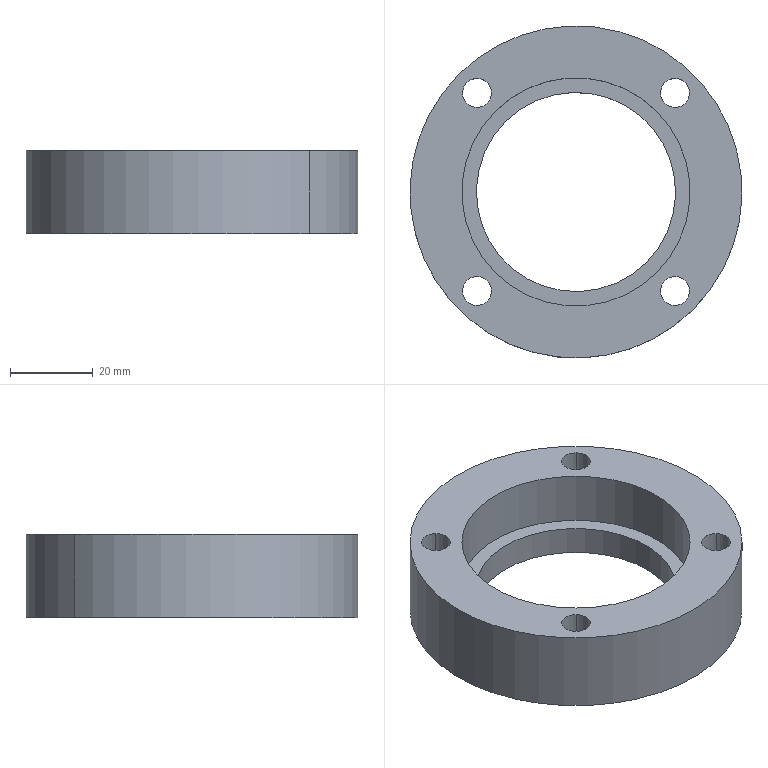Component | SolidWorks | 6006BearingHousing-3 | 1 solid | 29 faces | box 80 x 80 x 20 mm | volume 52542 mm3 | cylinder 22 | plane 7 | commonest cylinder face diameters 11 x8 7 x8 80 x2 55 x2 48 x2
STEP:
#1=COLOUR_RGB('',0.7922,0.8196,0.9333);
#2=FILL_AREA_STYLE_COLOUR('',#1);
#3=FILL_AREA_STYLE('',(#2));
#4=SURFACE_STYLE_FILL_AREA(#3);
#5=SURFACE_SIDE_STYLE('',(#4));
#6=SURFACE_STYLE_USAGE(.BOTH.,#5);
#7=PRESENTATION_STYLE_ASSIGNMENT((#6));
#8=CARTESIAN_POINT('',(7.284,48.013,-3.898));
#9=VERTEX_POINT('',#8);
#10=CARTESIAN_POINT('',(6.978,47.707,-3.898));
#11=VERTEX_POINT('',#10);
#12=CARTESIAN_POINT('',(7.131,47.86,-3.898));
#13=DIRECTION('',(0.,0.,-1.));
#14=DIRECTION('',(-0.7071,-0.7071,0.));
#15=AXIS2_PLACEMENT_3D('',#12,#13,#14);
#16=CIRCLE('',#15,0.2165);
#17=EDGE_CURVE('',#9,#11,#16,.T.);
#18=ORIENTED_EDGE('',*,*,#17,.F.);
#19=CARTESIAN_POINT('',(7.284,48.013,-4.134));
#20=VERTEX_POINT('',#19);
#21=CARTESIAN_POINT('',(7.284,48.013,-4.134));
#22=DIRECTION('',(0.,0.,-1.));
#23=VECTOR('',#22,39.37);
#24=LINE('',#21,#23);
#25=EDGE_CURVE('',#9,#20,#24,.T.);
#26=ORIENTED_EDGE('',*,*,#25,.T.);
#27=CARTESIAN_POINT('',(6.978,47.707,-4.134));
#28=VERTEX_POINT('',#27);
#29=CARTESIAN_POINT('',(7.131,47.86,-4.134));
#30=DIRECTION('',(0.,0.,-1.));
#31=DIRECTION('',(-0.7071,-0.7071,0.));
#32=AXIS2_PLACEMENT_3D('',#29,#30,#31);
#33=CIRCLE('',#32,0.2165);
#34=EDGE_CURVE('',#20,#28,#33,.T.);
#35=ORIENTED_EDGE('',*,*,#34,.T.);
#36=CARTESIAN_POINT('',(6.978,47.707,-4.134));
#37=DIRECTION('',(0.,0.,-1.));
#38=VECTOR('',#37,39.37);
#39=LINE('',#36,#38);
#40=EDGE_CURVE('',#11,#28,#39,.T.);
#41=ORIENTED_EDGE('',*,*,#40,.F.);
#42=EDGE_LOOP('',(#18,#26,#35,#41));
#43=FACE_OUTER_BOUND('',#42,.T.);
#44=CARTESIAN_POINT('',(7.131,47.86,-4.134));
#45=DIRECTION('',(0.,0.,-1.));
#46=DIRECTION('',(-0.7071,-0.7071,0.));
#47=AXIS2_PLACEMENT_3D('',#44,#45,#46);
#48=CYLINDRICAL_SURFACE('',#47,0.2165);
#49=ADVANCED_FACE('',(#43),#48,.F.);
#50=CARTESIAN_POINT('',(7.229,47.957,-3.346));
#51=VERTEX_POINT('',#50);
#52=CARTESIAN_POINT('',(7.034,47.762,-3.346));
#53=VERTEX_POINT('',#52);
#54=CARTESIAN_POINT('',(7.131,47.86,-3.346));
#55=DIRECTION('',(0.,0.,-1.));
#56=DIRECTION('',(-0.7071,-0.7071,0.));
#57=AXIS2_PLACEMENT_3D('',#54,#55,#56);
#58=CIRCLE('',#57,0.1378);
#59=EDGE_CURVE('',#51,#53,#58,.T.);
#60=ORIENTED_EDGE('',*,*,#59,.F.);
#61=CARTESIAN_POINT('',(7.229,47.957,-3.898));
#62=VERTEX_POINT('',#61);
#63=CARTESIAN_POINT('',(7.229,47.957,-4.134));
#64=DIRECTION('',(0.,0.,-1.));
#65=VECTOR('',#64,39.37);
#66=LINE('',#63,#65);
#67=EDGE_CURVE('',#51,#62,#66,.T.);
#68=ORIENTED_EDGE('',*,*,#67,.T.);
#69=CARTESIAN_POINT('',(7.034,47.762,-3.898));
#70=VERTEX_POINT('',#69);
#71=CARTESIAN_POINT('',(7.131,47.86,-3.898));
#72=DIRECTION('',(0.,0.,-1.));
#73=DIRECTION('',(-0.7071,-0.7071,0.));
#74=AXIS2_PLACEMENT_3D('',#71,#72,#73);
#75=CIRCLE('',#74,0.1378);
#76=EDGE_CURVE('',#62,#70,#75,.T.);
#77=ORIENTED_EDGE('',*,*,#76,.T.);
#78=CARTESIAN_POINT('',(7.034,47.762,-4.134));
#79=DIRECTION('',(0.,0.,-1.));
#80=VECTOR('',#79,39.37);
#81=LINE('',#78,#80);
#82=EDGE_CURVE('',#53,#70,#81,.T.);
#83=ORIENTED_EDGE('',*,*,#82,.F.);
#84=EDGE_LOOP('',(#60,#68,#77,#83));
#85=FACE_OUTER_BOUND('',#84,.T.);
#86=CARTESIAN_POINT('',(7.131,47.86,-4.134));
#87=DIRECTION('',(0.,0.,-1.));
#88=DIRECTION('',(-0.7071,-0.7071,0.));
#89=AXIS2_PLACEMENT_3D('',#86,#87,#88);
#90=CYLINDRICAL_SURFACE('',#89,0.1378);
#91=ADVANCED_FACE('',(#85),#90,.F.);
#92=CARTESIAN_POINT('',(7.284,49.892,-3.898));
#93=VERTEX_POINT('',#92);
#94=CARTESIAN_POINT('',(6.978,49.586,-3.898));
#95=VERTEX_POINT('',#94);
#96=CARTESIAN_POINT('',(7.131,49.739,-3.898));
#97=DIRECTION('',(0.,0.,-1.));
#98=DIRECTION('',(-0.7071,-0.7071,0.));
#99=AXIS2_PLACEMENT_3D('',#96,#97,#98);
#100=CIRCLE('',#99,0.2165);
#101=EDGE_CURVE('',#93,#95,#100,.T.);
#102=ORIENTED_EDGE('',*,*,#101,.F.);
#103=CARTESIAN_POINT('',(7.284,49.892,-4.134));
#104=VERTEX_POINT('',#103);
#105=CARTESIAN_POINT('',(7.284,49.892,-4.134));
#106=DIRECTION('',(0.,0.,-1.));
#107=VECTOR('',#106,39.37);
#108=LINE('',#105,#107);
#109=EDGE_CURVE('',#93,#104,#108,.T.);
#110=ORIENTED_EDGE('',*,*,#109,.T.);
#111=CARTESIAN_POINT('',(6.978,49.586,-4.134));
#112=VERTEX_POINT('',#111);
#113=CARTESIAN_POINT('',(7.131,49.739,-4.134));
#114=DIRECTION('',(0.,0.,-1.));
#115=DIRECTION('',(-0.7071,-0.7071,0.));
#116=AXIS2_PLACEMENT_3D('',#113,#114,#115);
#117=CIRCLE('',#116,0.2165);
#118=EDGE_CURVE('',#104,#112,#117,.T.);
#119=ORIENTED_EDGE('',*,*,#118,.T.);
#120=CARTESIAN_POINT('',(6.978,49.586,-4.134));
#121=DIRECTION('',(0.,0.,-1.));
#122=VECTOR('',#121,39.37);
#123=LINE('',#120,#122);
#124=EDGE_CURVE('',#95,#112,#123,.T.);
#125=ORIENTED_EDGE('',*,*,#124,.F.);
#126=EDGE_LOOP('',(#102,#110,#119,#125));
#127=FACE_OUTER_BOUND('',#126,.T.);
#128=CARTESIAN_POINT('',(7.131,49.739,-4.134));
#129=DIRECTION('',(0.,0.,-1.));
#130=DIRECTION('',(-0.7071,-0.7071,0.));
#131=AXIS2_PLACEMENT_3D('',#128,#129,#130);
#132=CYLINDRICAL_SURFACE('',#131,0.2165);
#133=ADVANCED_FACE('',(#127),#132,.F.);
#134=CARTESIAN_POINT('',(7.229,49.836,-3.346));
#135=VERTEX_POINT('',#134);
#136=CARTESIAN_POINT('',(7.034,49.641,-3.346));
#137=VERTEX_POINT('',#136);
#138=CARTESIAN_POINT('',(7.131,49.739,-3.346));
#139=DIRECTION('',(0.,0.,-1.));
#140=DIRECTION('',(-0.7071,-0.7071,0.));
#141=AXIS2_PLACEMENT_3D('',#138,#139,#140);
#142=CIRCLE('',#141,0.1378);
#143=EDGE_CURVE('',#135,#137,#142,.T.);
#144=ORIENTED_EDGE('',*,*,#143,.F.);
#145=CARTESIAN_POINT('',(7.229,49.836,-3.898));
#146=VERTEX_POINT('',#145);
#147=CARTESIAN_POINT('',(7.229,49.836,-4.134));
#148=DIRECTION('',(0.,0.,-1.));
#149=VECTOR('',#148,39.37);
#150=LINE('',#147,#149);
#151=EDGE_CURVE('',#135,#146,#150,.T.);
#152=ORIENTED_EDGE('',*,*,#151,.T.);
#153=CARTESIAN_POINT('',(7.034,49.641,-3.898));
#154=VERTEX_POINT('',#153);
#155=CARTESIAN_POINT('',(7.131,49.739,-3.898));
#156=DIRECTION('',(0.,0.,-1.));
#157=DIRECTION('',(-0.7071,-0.7071,0.));
#158=AXIS2_PLACEMENT_3D('',#155,#156,#157);
#159=CIRCLE('',#158,0.1378);
#160=EDGE_CURVE('',#146,#154,#159,.T.);
#161=ORIENTED_EDGE('',*,*,#160,.T.);
#162=CARTESIAN_POINT('',(7.034,49.641,-4.134));
#163=DIRECTION('',(0.,0.,-1.));
#164=VECTOR('',#163,39.37);
#165=LINE('',#162,#164);
#166=EDGE_CURVE('',#137,#154,#165,.T.);
#167=ORIENTED_EDGE('',*,*,#166,.F.);
#168=EDGE_LOOP('',(#144,#152,#161,#167));
#169=FACE_OUTER_BOUND('',#168,.T.);
#170=CARTESIAN_POINT('',(7.131,49.739,-4.134));
#171=DIRECTION('',(0.,0.,-1.));
#172=DIRECTION('',(-0.7071,-0.7071,0.));
#173=AXIS2_PLACEMENT_3D('',#170,#171,#172);
#174=CYLINDRICAL_SURFACE('',#173,0.1378);
#175=ADVANCED_FACE('',(#169),#174,.F.);
#176=CARTESIAN_POINT('',(9.164,48.013,-3.898));
#177=VERTEX_POINT('',#176);
#178=CARTESIAN_POINT('',(8.857,47.707,-3.898));
#179=VERTEX_POINT('',#178);
#180=CARTESIAN_POINT('',(9.01,47.86,-3.898));
#181=DIRECTION('',(0.,0.,-1.));
#182=DIRECTION('',(-0.7071,-0.7071,0.));
#183=AXIS2_PLACEMENT_3D('',#180,#181,#182);
#184=CIRCLE('',#183,0.2165);
#185=EDGE_CURVE('',#177,#179,#184,.T.);
#186=ORIENTED_EDGE('',*,*,#185,.F.);
#187=CARTESIAN_POINT('',(9.164,48.013,-4.134));
#188=VERTEX_POINT('',#187);
#189=CARTESIAN_POINT('',(9.164,48.013,-4.134));
#190=DIRECTION('',(0.,0.,-1.));
#191=VECTOR('',#190,39.37);
#192=LINE('',#189,#191);
#193=EDGE_CURVE('',#177,#188,#192,.T.);
#194=ORIENTED_EDGE('',*,*,#193,.T.);
#195=CARTESIAN_POINT('',(8.857,47.707,-4.134));
#196=VERTEX_POINT('',#195);
#197=CARTESIAN_POINT('',(9.01,47.86,-4.134));
#198=DIRECTION('',(0.,0.,-1.));
#199=DIRECTION('',(-0.7071,-0.7071,0.));
#200=AXIS2_PLACEMENT_3D('',#197,#198,#199);
#201=CIRCLE('',#200,0.2165);
#202=EDGE_CURVE('',#188,#196,#201,.T.);
#203=ORIENTED_EDGE('',*,*,#202,.T.);
#204=CARTESIAN_POINT('',(8.857,47.707,-4.134));
#205=DIRECTION('',(0.,0.,-1.));
#206=VECTOR('',#205,39.37);
#207=LINE('',#204,#206);
#208=EDGE_CURVE('',#179,#196,#207,.T.);
#209=ORIENTED_EDGE('',*,*,#208,.F.);
#210=EDGE_LOOP('',(#186,#194,#203,#209));
#211=FACE_OUTER_BOUND('',#210,.T.);
#212=CARTESIAN_POINT('',(9.01,47.86,-4.134));
#213=DIRECTION('',(0.,0.,-1.));
#214=DIRECTION('',(-0.7071,-0.7071,0.));
#215=AXIS2_PLACEMENT_3D('',#212,#213,#214);
#216=CYLINDRICAL_SURFACE('',#215,0.2165);
#217=ADVANCED_FACE('',(#211),#216,.F.);
#218=CARTESIAN_POINT('',(9.108,47.957,-3.346));
#219=VERTEX_POINT('',#218);
#220=CARTESIAN_POINT('',(8.913,47.762,-3.346));
#221=VERTEX_POINT('',#220);
#222=CARTESIAN_POINT('',(9.01,47.86,-3.346));
#223=DIRECTION('',(0.,0.,-1.));
#224=DIRECTION('',(-0.7071,-0.7071,0.));
#225=AXIS2_PLACEMENT_3D('',#222,#223,#224);
#226=CIRCLE('',#225,0.1378);
#227=EDGE_CURVE('',#219,#221,#226,.T.);
#228=ORIENTED_EDGE('',*,*,#227,.F.);
#229=CARTESIAN_POINT('',(9.108,47.957,-3.898));
#230=VERTEX_POINT('',#229);
#231=CARTESIAN_POINT('',(9.108,47.957,-4.134));
#232=DIRECTION('',(0.,0.,-1.));
#233=VECTOR('',#232,39.37);
#234=LINE('',#231,#233);
#235=EDGE_CURVE('',#219,#230,#234,.T.);
#236=ORIENTED_EDGE('',*,*,#235,.T.);
#237=CARTESIAN_POINT('',(8.913,47.762,-3.898));
#238=VERTEX_POINT('',#237);
#239=CARTESIAN_POINT('',(9.01,47.86,-3.898));
#240=DIRECTION('',(0.,0.,-1.));
#241=DIRECTION('',(-0.7071,-0.7071,0.));
#242=AXIS2_PLACEMENT_3D('',#239,#240,#241);
#243=CIRCLE('',#242,0.1378);
#244=EDGE_CURVE('',#230,#238,#243,.T.);
#245=ORIENTED_EDGE('',*,*,#244,.T.);
#246=CARTESIAN_POINT('',(8.913,47.762,-4.134));
#247=DIRECTION('',(0.,0.,-1.));
#248=VECTOR('',#247,39.37);
#249=LINE('',#246,#248);
#250=EDGE_CURVE('',#221,#238,#249,.T.);
#251=ORIENTED_EDGE('',*,*,#250,.F.);
#252=EDGE_LOOP('',(#228,#236,#245,#251));
#253=FACE_OUTER_BOUND('',#252,.T.);
#254=CARTESIAN_POINT('',(9.01,47.86,-4.134));
#255=DIRECTION('',(0.,0.,-1.));
#256=DIRECTION('',(-0.7071,-0.7071,0.));
#257=AXIS2_PLACEMENT_3D('',#254,#255,#256);
#258=CYLINDRICAL_SURFACE('',#257,0.1378);
#259=ADVANCED_FACE('',(#253),#258,.F.);
#260=CARTESIAN_POINT('',(9.164,49.892,-3.898));
#261=VERTEX_POINT('',#260);
#262=CARTESIAN_POINT('',(8.857,49.586,-3.898));
#263=VERTEX_POINT('',#262);
#264=CARTESIAN_POINT('',(9.01,49.739,-3.898));
#265=DIRECTION('',(0.,0.,-1.));
#266=DIRECTION('',(-0.7071,-0.7071,0.));
#267=AXIS2_PLACEMENT_3D('',#264,#265,#266);
#268=CIRCLE('',#267,0.2165);
#269=EDGE_CURVE('',#261,#263,#268,.T.);
#270=ORIENTED_EDGE('',*,*,#269,.F.);
#271=CARTESIAN_POINT('',(9.164,49.892,-4.134));
#272=VERTEX_POINT('',#271);
#273=CARTESIAN_POINT('',(9.164,49.892,-4.134));
#274=DIRECTION('',(0.,0.,-1.));
#275=VECTOR('',#274,39.37);
#276=LINE('',#273,#275);
#277=EDGE_CURVE('',#261,#272,#276,.T.);
#278=ORIENTED_EDGE('',*,*,#277,.T.);
#279=CARTESIAN_POINT('',(8.857,49.586,-4.134));
#280=VERTEX_POINT('',#279);
#281=CARTESIAN_POINT('',(9.01,49.739,-4.134));
#282=DIRECTION('',(0.,0.,-1.));
#283=DIRECTION('',(-0.7071,-0.7071,0.));
#284=AXIS2_PLACEMENT_3D('',#281,#282,#283);
#285=CIRCLE('',#284,0.2165);
#286=EDGE_CURVE('',#272,#280,#285,.T.);
#287=ORIENTED_EDGE('',*,*,#286,.T.);
#288=CARTESIAN_POINT('',(8.857,49.586,-4.134));
#289=DIRECTION('',(0.,0.,-1.));
#290=VECTOR('',#289,39.37);
#291=LINE('',#288,#290);
#292=EDGE_CURVE('',#263,#280,#291,.T.);
#293=ORIENTED_EDGE('',*,*,#292,.F.);
#294=EDGE_LOOP('',(#270,#278,#287,#293));
#295=FACE_OUTER_BOUND('',#294,.T.);
#296=CARTESIAN_POINT('',(9.01,49.739,-4.134));
#297=DIRECTION('',(0.,0.,-1.));
#298=DIRECTION('',(-0.7071,-0.7071,0.));
#299=AXIS2_PLACEMENT_3D('',#296,#297,#298);
#300=CYLINDRICAL_SURFACE('',#299,0.2165);
#301=ADVANCED_FACE('',(#295),#300,.F.);
#302=CARTESIAN_POINT('',(9.108,49.836,-3.346));
#303=VERTEX_POINT('',#302);
#304=CARTESIAN_POINT('',(8.913,49.641,-3.346));
#305=VERTEX_POINT('',#304);
#306=CARTESIAN_POINT('',(9.01,49.739,-3.346));
#307=DIRECTION('',(0.,0.,-1.));
#308=DIRECTION('',(-0.7071,-0.7071,0.));
#309=AXIS2_PLACEMENT_3D('',#306,#307,#308);
#310=CIRCLE('',#309,0.1378);
#311=EDGE_CURVE('',#303,#305,#310,.T.);
#312=ORIENTED_EDGE('',*,*,#311,.F.);
#313=CARTESIAN_POINT('',(9.108,49.836,-3.898));
#314=VERTEX_POINT('',#313);
#315=CARTESIAN_POINT('',(9.108,49.836,-4.134));
#316=DIRECTION('',(0.,0.,-1.));
#317=VECTOR('',#316,39.37);
#318=LINE('',#315,#317);
#319=EDGE_CURVE('',#303,#314,#318,.T.);
#320=ORIENTED_EDGE('',*,*,#319,.T.);
#321=CARTESIAN_POINT('',(8.913,49.641,-3.898));
#322=VERTEX_POINT('',#321);
#323=CARTESIAN_POINT('',(9.01,49.739,-3.898));
#324=DIRECTION('',(0.,0.,-1.));
#325=DIRECTION('',(-0.7071,-0.7071,0.));
#326=AXIS2_PLACEMENT_3D('',#323,#324,#325);
#327=CIRCLE('',#326,0.1378);
#328=EDGE_CURVE('',#314,#322,#327,.T.);
#329=ORIENTED_EDGE('',*,*,#328,.T.);
#330=CARTESIAN_POINT('',(8.913,49.641,-4.134));
#331=DIRECTION('',(0.,0.,-1.));
#332=VECTOR('',#331,39.37);
#333=LINE('',#330,#332);
#334=EDGE_CURVE('',#305,#322,#333,.T.);
#335=ORIENTED_EDGE('',*,*,#334,.F.);
#336=EDGE_LOOP('',(#312,#320,#329,#335));
#337=FACE_OUTER_BOUND('',#336,.T.);
#338=CARTESIAN_POINT('',(9.01,49.739,-4.134));
#339=DIRECTION('',(0.,0.,-1.));
#340=DIRECTION('',(-0.7071,-0.7071,0.));
#341=AXIS2_PLACEMENT_3D('',#338,#339,#340);
#342=CYLINDRICAL_SURFACE('',#341,0.1378);
#343=ADVANCED_FACE('',(#337),#342,.F.);
#344=CARTESIAN_POINT('',(6.957,49.913,-3.346));
#345=VERTEX_POINT('',#344);
#346=CARTESIAN_POINT('',(9.184,47.686,-3.346));
#347=VERTEX_POINT('',#346);
#348=CARTESIAN_POINT('',(8.071,48.799,-3.346));
#349=DIRECTION('',(-0.,0.,-1.));
#350=DIRECTION('',(-0.7071,0.7071,0.));
#351=AXIS2_PLACEMENT_3D('',#348,#349,#350);
#352=CIRCLE('',#351,1.575);
#353=EDGE_CURVE('',#345,#347,#352,.T.);
#354=ORIENTED_EDGE('',*,*,#353,.T.);
#355=CARTESIAN_POINT('',(9.184,47.686,-4.134));
#356=VERTEX_POINT('',#355);
#357=CARTESIAN_POINT('',(9.184,47.686,-24.446));
#358=DIRECTION('',(-0.,0.,-1.));
#359=VECTOR('',#358,39.37);
#360=LINE('',#357,#359);
#361=EDGE_CURVE('',#347,#356,#360,.T.);
#362=ORIENTED_EDGE('',*,*,#361,.T.);
#363=CARTESIAN_POINT('',(6.957,49.913,-4.134));
#364=VERTEX_POINT('',#363);
#365=CARTESIAN_POINT('',(8.071,48.799,-4.134));
#366=DIRECTION('',(-0.,0.,-1.));
#367=DIRECTION('',(-0.7071,0.7071,0.));
#368=AXIS2_PLACEMENT_3D('',#365,#366,#367);
#369=CIRCLE('',#368,1.575);
#370=EDGE_CURVE('',#364,#356,#369,.T.);
#371=ORIENTED_EDGE('',*,*,#370,.F.);
#372=CARTESIAN_POINT('',(6.957,49.913,-24.446));
#373=DIRECTION('',(-0.,0.,-1.));
#374=VECTOR('',#373,39.37);
#375=LINE('',#372,#374);
#376=EDGE_CURVE('',#345,#364,#375,.T.);
#377=ORIENTED_EDGE('',*,*,#376,.F.);
#378=EDGE_LOOP('',(#354,#362,#371,#377));
#379=FACE_OUTER_BOUND('',#378,.T.);
#380=CARTESIAN_POINT('',(8.071,48.799,-24.446));
#381=DIRECTION('',(-0.,0.,-1.));
#382=DIRECTION('',(-0.7071,0.7071,0.));
#383=AXIS2_PLACEMENT_3D('',#380,#381,#382);
#384=CYLINDRICAL_SURFACE('',#383,1.575);
#385=ADVANCED_FACE('',(#379),#384,.T.);
#386=CARTESIAN_POINT('',(8.836,48.034,-3.346));
#387=VERTEX_POINT('',#386);
#388=CARTESIAN_POINT('',(7.305,49.565,-3.346));
#389=VERTEX_POINT('',#388);
#390=CARTESIAN_POINT('',(8.071,48.799,-3.346));
#391=DIRECTION('',(-0.,0.,-1.));
#392=DIRECTION('',(-0.7071,0.7071,0.));
#393=AXIS2_PLACEMENT_3D('',#390,#391,#392);
#394=CIRCLE('',#393,1.083);
#395=EDGE_CURVE('',#387,#389,#394,.T.);
#396=ORIENTED_EDGE('',*,*,#395,.F.);
#397=CARTESIAN_POINT('',(8.836,48.034,-3.858));
#398=VERTEX_POINT('',#397);
#399=CARTESIAN_POINT('',(8.836,48.034,-24.446));
#400=DIRECTION('',(-0.,0.,-1.));
#401=VECTOR('',#400,39.37);
#402=LINE('',#399,#401);
#403=EDGE_CURVE('',#387,#398,#402,.T.);
#404=ORIENTED_EDGE('',*,*,#403,.T.);
#405=CARTESIAN_POINT('',(7.305,49.565,-3.858));
#406=VERTEX_POINT('',#405);
#407=CARTESIAN_POINT('',(8.071,48.799,-3.858));
#408=DIRECTION('',(-0.,0.,-1.));
#409=DIRECTION('',(-0.7071,0.7071,0.));
#410=AXIS2_PLACEMENT_3D('',#407,#408,#409);
#411=CIRCLE('',#410,1.083);
#412=EDGE_CURVE('',#398,#406,#411,.T.);
#413=ORIENTED_EDGE('',*,*,#412,.T.);
#414=CARTESIAN_POINT('',(7.305,49.565,-24.446));
#415=DIRECTION('',(-0.,0.,-1.));
#416=VECTOR('',#415,39.37);
#417=LINE('',#414,#416);
#418=EDGE_CURVE('',#389,#406,#417,.T.);
#419=ORIENTED_EDGE('',*,*,#418,.F.);
#420=EDGE_LOOP('',(#396,#404,#413,#419));
#421=FACE_OUTER_BOUND('',#420,.T.);
#422=CARTESIAN_POINT('',(8.071,48.799,-24.446));
#423=DIRECTION('',(-0.,0.,-1.));
#424=DIRECTION('',(-0.7071,0.7071,0.));
#425=AXIS2_PLACEMENT_3D('',#422,#423,#424);
#426=CYLINDRICAL_SURFACE('',#425,1.083);
#427=ADVANCED_FACE('',(#421),#426,.F.);
#428=CARTESIAN_POINT('',(8.739,48.131,-3.858));
#429=VERTEX_POINT('',#428);
#430=CARTESIAN_POINT('',(7.403,49.467,-3.858));
#431=VERTEX_POINT('',#430);
#432=CARTESIAN_POINT('',(8.071,48.799,-3.858));
#433=DIRECTION('',(-0.,0.,-1.));
#434=DIRECTION('',(-0.7071,0.7071,0.));
#435=AXIS2_PLACEMENT_3D('',#432,#433,#434);
#436=CIRCLE('',#435,0.9449);
#437=EDGE_CURVE('',#429,#431,#436,.T.);
#438=ORIENTED_EDGE('',*,*,#437,.F.);
#439=CARTESIAN_POINT('',(8.739,48.131,-4.134));
#440=VERTEX_POINT('',#439);
#441=CARTESIAN_POINT('',(8.739,48.131,-24.446));
#442=DIRECTION('',(-0.,0.,-1.));
#443=VECTOR('',#442,39.37);
#444=LINE('',#441,#443);
#445=EDGE_CURVE('',#429,#440,#444,.T.);
#446=ORIENTED_EDGE('',*,*,#445,.T.);
#447=CARTESIAN_POINT('',(7.403,49.467,-4.134));
#448=VERTEX_POINT('',#447);
#449=CARTESIAN_POINT('',(8.071,48.799,-4.134));
#450=DIRECTION('',(-0.,0.,-1.));
#451=DIRECTION('',(-0.7071,0.7071,0.));
#452=AXIS2_PLACEMENT_3D('',#449,#450,#451);
#453=CIRCLE('',#452,0.9449);
#454=EDGE_CURVE('',#440,#448,#453,.T.);
#455=ORIENTED_EDGE('',*,*,#454,.T.);
#456=CARTESIAN_POINT('',(7.403,49.467,-24.446));
#457=DIRECTION('',(-0.,0.,-1.));
#458=VECTOR('',#457,39.37);
#459=LINE('',#456,#458);
#460=EDGE_CURVE('',#431,#448,#459,.T.);
#461=ORIENTED_EDGE('',*,*,#460,.F.);
#462=EDGE_LOOP('',(#438,#446,#455,#461));
#463=FACE_OUTER_BOUND('',#462,.T.);
#464=CARTESIAN_POINT('',(8.071,48.799,-24.446));
#465=DIRECTION('',(-0.,0.,-1.));
#466=DIRECTION('',(-0.7071,0.7071,0.));
#467=AXIS2_PLACEMENT_3D('',#464,#465,#466);
#468=CYLINDRICAL_SURFACE('',#467,0.9449);
#469=ADVANCED_FACE('',(#463),#468,.F.);
#470=CARTESIAN_POINT('',(7.131,47.86,-4.134));
#471=DIRECTION('',(0.,0.,-1.));
#472=DIRECTION('',(-0.7071,-0.7071,0.));
#473=AXIS2_PLACEMENT_3D('',#470,#471,#472);
#474=CIRCLE('',#473,0.2165);
#475=EDGE_CURVE('',#28,#20,#474,.T.);
#476=ORIENTED_EDGE('',*,*,#475,.F.);
#477=ORIENTED_EDGE('',*,*,#34,.F.);
#478=EDGE_LOOP('',(#476,#477));
#479=FACE_BOUND('',#478,.T.);
#480=CARTESIAN_POINT('',(7.131,49.739,-4.134));
#481=DIRECTION('',(0.,0.,-1.));
#482=DIRECTION('',(-0.7071,-0.7071,0.));
#483=AXIS2_PLACEMENT_3D('',#480,#481,#482);
#484=CIRCLE('',#483,0.2165);
#485=EDGE_CURVE('',#112,#104,#484,.T.);
#486=ORIENTED_EDGE('',*,*,#485,.F.);
#487=ORIENTED_EDGE('',*,*,#118,.F.);
#488=EDGE_LOOP('',(#486,#487));
#489=FACE_BOUND('',#488,.T.);
#490=CARTESIAN_POINT('',(9.01,47.86,-4.134));
#491=DIRECTION('',(0.,0.,-1.));
#492=DIRECTION('',(-0.7071,-0.7071,0.));
#493=AXIS2_PLACEMENT_3D('',#490,#491,#492);
#494=CIRCLE('',#493,0.2165);
#495=EDGE_CURVE('',#196,#188,#494,.T.);
#496=ORIENTED_EDGE('',*,*,#495,.F.);
#497=ORIENTED_EDGE('',*,*,#202,.F.);
#498=EDGE_LOOP('',(#496,#497));
#499=FACE_BOUND('',#498,.T.);
#500=CARTESIAN_POINT('',(9.01,49.739,-4.134));
#501=DIRECTION('',(0.,0.,-1.));
#502=DIRECTION('',(-0.7071,-0.7071,0.));
#503=AXIS2_PLACEMENT_3D('',#500,#501,#502);
#504=CIRCLE('',#503,0.2165);
#505=EDGE_CURVE('',#280,#272,#504,.T.);
#506=ORIENTED_EDGE('',*,*,#505,.F.);
#507=ORIENTED_EDGE('',*,*,#286,.F.);
#508=EDGE_LOOP('',(#506,#507));
#509=FACE_BOUND('',#508,.T.);
#510=ORIENTED_EDGE('',*,*,#370,.T.);
#511=CARTESIAN_POINT('',(8.071,48.799,-4.134));
#512=DIRECTION('',(-0.,0.,-1.));
#513=DIRECTION('',(-0.7071,0.7071,0.));
#514=AXIS2_PLACEMENT_3D('',#511,#512,#513);
#515=CIRCLE('',#514,1.575);
#516=EDGE_CURVE('',#356,#364,#515,.T.);
#517=ORIENTED_EDGE('',*,*,#516,.T.);
#518=EDGE_LOOP('',(#510,#517));
#519=FACE_OUTER_BOUND('',#518,.T.);
#520=CARTESIAN_POINT('',(8.071,48.799,-4.134));
#521=DIRECTION('',(-0.,0.,-1.));
#522=DIRECTION('',(-0.7071,0.7071,0.));
#523=AXIS2_PLACEMENT_3D('',#520,#521,#522);
#524=CIRCLE('',#523,0.9449);
#525=EDGE_CURVE('',#448,#440,#524,.T.);
#526=ORIENTED_EDGE('',*,*,#525,.F.);
#527=ORIENTED_EDGE('',*,*,#454,.F.);
#528=EDGE_LOOP('',(#526,#527));
#529=FACE_BOUND('',#528,.T.);
#530=CARTESIAN_POINT('',(6.957,49.913,-4.134));
#531=DIRECTION('',(-0.,0.,-1.));
#532=DIRECTION('',(-0.7071,0.7071,0.));
#533=AXIS2_PLACEMENT_3D('',#530,#531,#532);
#534=PLANE('',#533);
#535=ADVANCED_FACE('',(#479,#489,#499,#509,#519,#529),#534,.T.);
#536=ORIENTED_EDGE('',*,*,#445,.F.);
#537=CARTESIAN_POINT('',(8.071,48.799,-3.858));
#538=DIRECTION('',(-0.,0.,-1.));
#539=DIRECTION('',(-0.7071,0.7071,0.));
#540=AXIS2_PLACEMENT_3D('',#537,#538,#539);
#541=CIRCLE('',#540,0.9449);
#542=EDGE_CURVE('',#431,#429,#541,.T.);
#543=ORIENTED_EDGE('',*,*,#542,.F.);
#544=ORIENTED_EDGE('',*,*,#460,.T.);
#545=ORIENTED_EDGE('',*,*,#525,.T.);
#546=EDGE_LOOP('',(#536,#543,#544,#545));
#547=FACE_OUTER_BOUND('',#546,.T.);
#548=CARTESIAN_POINT('',(8.071,48.799,-24.446));
#549=DIRECTION('',(-0.,0.,-1.));
#550=DIRECTION('',(-0.7071,0.7071,0.));
#551=AXIS2_PLACEMENT_3D('',#548,#549,#550);
#552=CYLINDRICAL_SURFACE('',#551,0.9449);
#553=ADVANCED_FACE('',(#547),#552,.F.);
#554=ORIENTED_EDGE('',*,*,#542,.T.);
#555=ORIENTED_EDGE('',*,*,#437,.T.);
#556=EDGE_LOOP('',(#554,#555));
#557=FACE_BOUND('',#556,.T.);
#558=CARTESIAN_POINT('',(8.071,48.799,-3.858));
#559=DIRECTION('',(-0.,0.,-1.));
#560=DIRECTION('',(-0.7071,0.7071,0.));
#561=AXIS2_PLACEMENT_3D('',#558,#559,#560);
#562=CIRCLE('',#561,1.083);
#563=EDGE_CURVE('',#406,#398,#562,.T.);
#564=ORIENTED_EDGE('',*,*,#563,.F.);
#565=ORIENTED_EDGE('',*,*,#412,.F.);
#566=EDGE_LOOP('',(#564,#565));
#567=FACE_OUTER_BOUND('',#566,.T.);
#568=CARTESIAN_POINT('',(7.403,49.467,-3.858));
#569=DIRECTION('',(0.,-0.,1.));
#570=DIRECTION('',(0.7071,-0.7071,-0.));
#571=AXIS2_PLACEMENT_3D('',#568,#569,#570);
#572=PLANE('',#571);
#573=ADVANCED_FACE('',(#557,#567),#572,.T.);
#574=ORIENTED_EDGE('',*,*,#403,.F.);
#575=CARTESIAN_POINT('',(8.071,48.799,-3.346));
#576=DIRECTION('',(-0.,0.,-1.));
#577=DIRECTION('',(-0.7071,0.7071,0.));
#578=AXIS2_PLACEMENT_3D('',#575,#576,#577);
#579=CIRCLE('',#578,1.083);
#580=EDGE_CURVE('',#389,#387,#579,.T.);
#581=ORIENTED_EDGE('',*,*,#580,.F.);
#582=ORIENTED_EDGE('',*,*,#418,.T.);
#583=ORIENTED_EDGE('',*,*,#563,.T.);
#584=EDGE_LOOP('',(#574,#581,#582,#583));
#585=FACE_OUTER_BOUND('',#584,.T.);
#586=CARTESIAN_POINT('',(8.071,48.799,-24.446));
#587=DIRECTION('',(-0.,0.,-1.));
#588=DIRECTION('',(-0.7071,0.7071,0.));
#589=AXIS2_PLACEMENT_3D('',#586,#587,#588);
#590=CYLINDRICAL_SURFACE('',#589,1.083);
#591=ADVANCED_FACE('',(#585),#590,.F.);
#592=CARTESIAN_POINT('',(7.131,47.86,-3.346));
#593=DIRECTION('',(0.,0.,-1.));
#594=DIRECTION('',(-0.7071,-0.7071,0.));
#595=AXIS2_PLACEMENT_3D('',#592,#593,#594);
#596=CIRCLE('',#595,0.1378);
#597=EDGE_CURVE('',#53,#51,#596,.T.);
#598=ORIENTED_EDGE('',*,*,#597,.T.);
#599=ORIENTED_EDGE('',*,*,#59,.T.);
#600=EDGE_LOOP('',(#598,#599));
#601=FACE_BOUND('',#600,.T.);
#602=CARTESIAN_POINT('',(7.131,49.739,-3.346));
#603=DIRECTION('',(0.,0.,-1.));
#604=DIRECTION('',(-0.7071,-0.7071,0.));
#605=AXIS2_PLACEMENT_3D('',#602,#603,#604);
#606=CIRCLE('',#605,0.1378);
#607=EDGE_CURVE('',#137,#135,#606,.T.);
#608=ORIENTED_EDGE('',*,*,#607,.T.);
#609=ORIENTED_EDGE('',*,*,#143,.T.);
#610=EDGE_LOOP('',(#608,#609));
#611=FACE_BOUND('',#610,.T.);
#612=CARTESIAN_POINT('',(9.01,47.86,-3.346));
#613=DIRECTION('',(0.,0.,-1.));
#614=DIRECTION('',(-0.7071,-0.7071,0.));
#615=AXIS2_PLACEMENT_3D('',#612,#613,#614);
#616=CIRCLE('',#615,0.1378);
#617=EDGE_CURVE('',#221,#219,#616,.T.);
#618=ORIENTED_EDGE('',*,*,#617,.T.);
#619=ORIENTED_EDGE('',*,*,#227,.T.);
#620=EDGE_LOOP('',(#618,#619));
#621=FACE_BOUND('',#620,.T.);
#622=CARTESIAN_POINT('',(9.01,49.739,-3.346));
#623=DIRECTION('',(0.,0.,-1.));
#624=DIRECTION('',(-0.7071,-0.7071,0.));
#625=AXIS2_PLACEMENT_3D('',#622,#623,#624);
#626=CIRCLE('',#625,0.1378);
#627=EDGE_CURVE('',#305,#303,#626,.T.);
#628=ORIENTED_EDGE('',*,*,#627,.T.);
#629=ORIENTED_EDGE('',*,*,#311,.T.);
#630=EDGE_LOOP('',(#628,#629));
#631=FACE_BOUND('',#630,.T.);
#632=ORIENTED_EDGE('',*,*,#580,.T.);
#633=ORIENTED_EDGE('',*,*,#395,.T.);
#634=EDGE_LOOP('',(#632,#633));
#635=FACE_BOUND('',#634,.T.);
#636=ORIENTED_EDGE('',*,*,#353,.F.);
#637=CARTESIAN_POINT('',(8.071,48.799,-3.346));
#638=DIRECTION('',(-0.,0.,-1.));
#639=DIRECTION('',(-0.7071,0.7071,0.));
#640=AXIS2_PLACEMENT_3D('',#637,#638,#639);
#641=CIRCLE('',#640,1.575);
#642=EDGE_CURVE('',#347,#345,#641,.T.);
#643=ORIENTED_EDGE('',*,*,#642,.F.);
#644=EDGE_LOOP('',(#636,#643));
#645=FACE_OUTER_BOUND('',#644,.T.);
#646=CARTESIAN_POINT('',(7.305,49.565,-3.346));
#647=DIRECTION('',(0.,-0.,1.));
#648=DIRECTION('',(0.7071,-0.7071,-0.));
#649=AXIS2_PLACEMENT_3D('',#646,#647,#648);
#650=PLANE('',#649);
#651=ADVANCED_FACE('',(#601,#611,#621,#631,#635,#645),#650,.T.);
#652=ORIENTED_EDGE('',*,*,#361,.F.);
#653=ORIENTED_EDGE('',*,*,#642,.T.);
#654=ORIENTED_EDGE('',*,*,#376,.T.);
#655=ORIENTED_EDGE('',*,*,#516,.F.);
#656=EDGE_LOOP('',(#652,#653,#654,#655));
#657=FACE_OUTER_BOUND('',#656,.T.);
#658=CARTESIAN_POINT('',(8.071,48.799,-24.446));
#659=DIRECTION('',(-0.,0.,-1.));
#660=DIRECTION('',(-0.7071,0.7071,0.));
#661=AXIS2_PLACEMENT_3D('',#658,#659,#660);
#662=CYLINDRICAL_SURFACE('',#661,1.575);
#663=ADVANCED_FACE('',(#657),#662,.T.);
#664=ORIENTED_EDGE('',*,*,#319,.F.);
#665=ORIENTED_EDGE('',*,*,#627,.F.);
#666=ORIENTED_EDGE('',*,*,#334,.T.);
#667=CARTESIAN_POINT('',(9.01,49.739,-3.898));
#668=DIRECTION('',(0.,0.,-1.));
#669=DIRECTION('',(-0.7071,-0.7071,0.));
#670=AXIS2_PLACEMENT_3D('',#667,#668,#669);
#671=CIRCLE('',#670,0.1378);
#672=EDGE_CURVE('',#322,#314,#671,.T.);
#673=ORIENTED_EDGE('',*,*,#672,.T.);
#674=EDGE_LOOP('',(#664,#665,#666,#673));
#675=FACE_OUTER_BOUND('',#674,.T.);
#676=CARTESIAN_POINT('',(9.01,49.739,-4.134));
#677=DIRECTION('',(0.,0.,-1.));
#678=DIRECTION('',(-0.7071,-0.7071,0.));
#679=AXIS2_PLACEMENT_3D('',#676,#677,#678);
#680=CYLINDRICAL_SURFACE('',#679,0.1378);
#681=ADVANCED_FACE('',(#675),#680,.F.);
#682=ORIENTED_EDGE('',*,*,#672,.F.);
#683=ORIENTED_EDGE('',*,*,#328,.F.);
#684=EDGE_LOOP('',(#682,#683));
#685=FACE_BOUND('',#684,.T.);
#686=CARTESIAN_POINT('',(9.01,49.739,-3.898));
#687=DIRECTION('',(0.,0.,-1.));
#688=DIRECTION('',(-0.7071,-0.7071,0.));
#689=AXIS2_PLACEMENT_3D('',#686,#687,#688);
#690=CIRCLE('',#689,0.2165);
#691=EDGE_CURVE('',#263,#261,#690,.T.);
#692=ORIENTED_EDGE('',*,*,#691,.T.);
#693=ORIENTED_EDGE('',*,*,#269,.T.);
#694=EDGE_LOOP('',(#692,#693));
#695=FACE_OUTER_BOUND('',#694,.T.);
#696=CARTESIAN_POINT('',(8.913,49.836,-3.898));
#697=DIRECTION('',(0.,-0.,1.));
#698=DIRECTION('',(0.7071,0.7071,0.));
#699=AXIS2_PLACEMENT_3D('',#696,#697,#698);
#700=PLANE('',#699);
#701=ADVANCED_FACE('',(#685,#695),#700,.F.);
#702=ORIENTED_EDGE('',*,*,#277,.F.);
#703=ORIENTED_EDGE('',*,*,#691,.F.);
#704=ORIENTED_EDGE('',*,*,#292,.T.);
#705=ORIENTED_EDGE('',*,*,#505,.T.);
#706=EDGE_LOOP('',(#702,#703,#704,#705));
#707=FACE_OUTER_BOUND('',#706,.T.);
#708=CARTESIAN_POINT('',(9.01,49.739,-4.134));
#709=DIRECTION('',(0.,0.,-1.));
#710=DIRECTION('',(-0.7071,-0.7071,0.));
#711=AXIS2_PLACEMENT_3D('',#708,#709,#710);
#712=CYLINDRICAL_SURFACE('',#711,0.2165);
#713=ADVANCED_FACE('',(#707),#712,.F.);
#714=ORIENTED_EDGE('',*,*,#235,.F.);
#715=ORIENTED_EDGE('',*,*,#617,.F.);
#716=ORIENTED_EDGE('',*,*,#250,.T.);
#717=CARTESIAN_POINT('',(9.01,47.86,-3.898));
#718=DIRECTION('',(0.,0.,-1.));
#719=DIRECTION('',(-0.7071,-0.7071,0.));
#720=AXIS2_PLACEMENT_3D('',#717,#718,#719);
#721=CIRCLE('',#720,0.1378);
#722=EDGE_CURVE('',#238,#230,#721,.T.);
#723=ORIENTED_EDGE('',*,*,#722,.T.);
#724=EDGE_LOOP('',(#714,#715,#716,#723));
#725=FACE_OUTER_BOUND('',#724,.T.);
#726=CARTESIAN_POINT('',(9.01,47.86,-4.134));
#727=DIRECTION('',(0.,0.,-1.));
#728=DIRECTION('',(-0.7071,-0.7071,0.));
#729=AXIS2_PLACEMENT_3D('',#726,#727,#728);
#730=CYLINDRICAL_SURFACE('',#729,0.1378);
#731=ADVANCED_FACE('',(#725),#730,.F.);
#732=ORIENTED_EDGE('',*,*,#722,.F.);
#733=ORIENTED_EDGE('',*,*,#244,.F.);
#734=EDGE_LOOP('',(#732,#733));
#735=FACE_BOUND('',#734,.T.);
#736=CARTESIAN_POINT('',(9.01,47.86,-3.898));
#737=DIRECTION('',(0.,0.,-1.));
#738=DIRECTION('',(-0.7071,-0.7071,0.));
#739=AXIS2_PLACEMENT_3D('',#736,#737,#738);
#740=CIRCLE('',#739,0.2165);
#741=EDGE_CURVE('',#179,#177,#740,.T.);
#742=ORIENTED_EDGE('',*,*,#741,.T.);
#743=ORIENTED_EDGE('',*,*,#185,.T.);
#744=EDGE_LOOP('',(#742,#743));
#745=FACE_OUTER_BOUND('',#744,.T.);
#746=CARTESIAN_POINT('',(8.913,47.957,-3.898));
#747=DIRECTION('',(0.,-0.,1.));
#748=DIRECTION('',(0.7071,0.7071,0.));
#749=AXIS2_PLACEMENT_3D('',#746,#747,#748);
#750=PLANE('',#749);
#751=ADVANCED_FACE('',(#735,#745),#750,.F.);
#752=ORIENTED_EDGE('',*,*,#193,.F.);
#753=ORIENTED_EDGE('',*,*,#741,.F.);
#754=ORIENTED_EDGE('',*,*,#208,.T.);
#755=ORIENTED_EDGE('',*,*,#495,.T.);
#756=EDGE_LOOP('',(#752,#753,#754,#755));
#757=FACE_OUTER_BOUND('',#756,.T.);
#758=CARTESIAN_POINT('',(9.01,47.86,-4.134));
#759=DIRECTION('',(0.,0.,-1.));
#760=DIRECTION('',(-0.7071,-0.7071,0.));
#761=AXIS2_PLACEMENT_3D('',#758,#759,#760);
#762=CYLINDRICAL_SURFACE('',#761,0.2165);
#763=ADVANCED_FACE('',(#757),#762,.F.);
#764=ORIENTED_EDGE('',*,*,#151,.F.);
#765=ORIENTED_EDGE('',*,*,#607,.F.);
#766=ORIENTED_EDGE('',*,*,#166,.T.);
#767=CARTESIAN_POINT('',(7.131,49.739,-3.898));
#768=DIRECTION('',(0.,0.,-1.));
#769=DIRECTION('',(-0.7071,-0.7071,0.));
#770=AXIS2_PLACEMENT_3D('',#767,#768,#769);
#771=CIRCLE('',#770,0.1378);
#772=EDGE_CURVE('',#154,#146,#771,.T.);
#773=ORIENTED_EDGE('',*,*,#772,.T.);
#774=EDGE_LOOP('',(#764,#765,#766,#773));
#775=FACE_OUTER_BOUND('',#774,.T.);
#776=CARTESIAN_POINT('',(7.131,49.739,-4.134));
#777=DIRECTION('',(0.,0.,-1.));
#778=DIRECTION('',(-0.7071,-0.7071,0.));
#779=AXIS2_PLACEMENT_3D('',#776,#777,#778);
#780=CYLINDRICAL_SURFACE('',#779,0.1378);
#781=ADVANCED_FACE('',(#775),#780,.F.);
#782=ORIENTED_EDGE('',*,*,#772,.F.);
#783=ORIENTED_EDGE('',*,*,#160,.F.);
#784=EDGE_LOOP('',(#782,#783));
#785=FACE_BOUND('',#784,.T.);
#786=CARTESIAN_POINT('',(7.131,49.739,-3.898));
#787=DIRECTION('',(0.,0.,-1.));
#788=DIRECTION('',(-0.7071,-0.7071,0.));
#789=AXIS2_PLACEMENT_3D('',#786,#787,#788);
#790=CIRCLE('',#789,0.2165);
#791=EDGE_CURVE('',#95,#93,#790,.T.);
#792=ORIENTED_EDGE('',*,*,#791,.T.);
#793=ORIENTED_EDGE('',*,*,#101,.T.);
#794=EDGE_LOOP('',(#792,#793));
#795=FACE_OUTER_BOUND('',#794,.T.);
#796=CARTESIAN_POINT('',(7.034,49.836,-3.898));
#797=DIRECTION('',(0.,-0.,1.));
#798=DIRECTION('',(0.7071,0.7071,0.));
#799=AXIS2_PLACEMENT_3D('',#796,#797,#798);
#800=PLANE('',#799);
#801=ADVANCED_FACE('',(#785,#795),#800,.F.);
#802=ORIENTED_EDGE('',*,*,#109,.F.);
#803=ORIENTED_EDGE('',*,*,#791,.F.);
#804=ORIENTED_EDGE('',*,*,#124,.T.);
#805=ORIENTED_EDGE('',*,*,#485,.T.);
#806=EDGE_LOOP('',(#802,#803,#804,#805));
#807=FACE_OUTER_BOUND('',#806,.T.);
#808=CARTESIAN_POINT('',(7.131,49.739,-4.134));
#809=DIRECTION('',(0.,0.,-1.));
#810=DIRECTION('',(-0.7071,-0.7071,0.));
#811=AXIS2_PLACEMENT_3D('',#808,#809,#810);
#812=CYLINDRICAL_SURFACE('',#811,0.2165);
#813=ADVANCED_FACE('',(#807),#812,.F.);
#814=ORIENTED_EDGE('',*,*,#67,.F.);
#815=ORIENTED_EDGE('',*,*,#597,.F.);
#816=ORIENTED_EDGE('',*,*,#82,.T.);
#817=CARTESIAN_POINT('',(7.131,47.86,-3.898));
#818=DIRECTION('',(0.,0.,-1.));
#819=DIRECTION('',(-0.7071,-0.7071,0.));
#820=AXIS2_PLACEMENT_3D('',#817,#818,#819);
#821=CIRCLE('',#820,0.1378);
#822=EDGE_CURVE('',#70,#62,#821,.T.);
#823=ORIENTED_EDGE('',*,*,#822,.T.);
#824=EDGE_LOOP('',(#814,#815,#816,#823));
#825=FACE_OUTER_BOUND('',#824,.T.);
#826=CARTESIAN_POINT('',(7.131,47.86,-4.134));
#827=DIRECTION('',(0.,0.,-1.));
#828=DIRECTION('',(-0.7071,-0.7071,0.));
#829=AXIS2_PLACEMENT_3D('',#826,#827,#828);
#830=CYLINDRICAL_SURFACE('',#829,0.1378);
#831=ADVANCED_FACE('',(#825),#830,.F.);
#832=ORIENTED_EDGE('',*,*,#822,.F.);
#833=ORIENTED_EDGE('',*,*,#76,.F.);
#834=EDGE_LOOP('',(#832,#833));
#835=FACE_BOUND('',#834,.T.);
#836=CARTESIAN_POINT('',(7.131,47.86,-3.898));
#837=DIRECTION('',(0.,0.,-1.));
#838=DIRECTION('',(-0.7071,-0.7071,0.));
#839=AXIS2_PLACEMENT_3D('',#836,#837,#838);
#840=CIRCLE('',#839,0.2165);
#841=EDGE_CURVE('',#11,#9,#840,.T.);
#842=ORIENTED_EDGE('',*,*,#841,.T.);
#843=ORIENTED_EDGE('',*,*,#17,.T.);
#844=EDGE_LOOP('',(#842,#843));
#845=FACE_OUTER_BOUND('',#844,.T.);
#846=CARTESIAN_POINT('',(7.034,47.957,-3.898));
#847=DIRECTION('',(0.,-0.,1.));
#848=DIRECTION('',(0.7071,0.7071,0.));
#849=AXIS2_PLACEMENT_3D('',#846,#847,#848);
#850=PLANE('',#849);
#851=ADVANCED_FACE('',(#835,#845),#850,.F.);
#852=ORIENTED_EDGE('',*,*,#25,.F.);
#853=ORIENTED_EDGE('',*,*,#841,.F.);
#854=ORIENTED_EDGE('',*,*,#40,.T.);
#855=ORIENTED_EDGE('',*,*,#475,.T.);
#856=EDGE_LOOP('',(#852,#853,#854,#855));
#857=FACE_OUTER_BOUND('',#856,.T.);
#858=CARTESIAN_POINT('',(7.131,47.86,-4.134));
#859=DIRECTION('',(0.,0.,-1.));
#860=DIRECTION('',(-0.7071,-0.7071,0.));
#861=AXIS2_PLACEMENT_3D('',#858,#859,#860);
#862=CYLINDRICAL_SURFACE('',#861,0.2165);
#863=ADVANCED_FACE('',(#857),#862,.F.);
#864=CLOSED_SHELL('',(#49,#91,#133,#175,#217,#259,#301,#343,#385,#427,#469,#535,#553,#573,#591,#651,#663,#681,#701,#713,#731,#751,#763,#781,#801,#813,#831,#851,#863));
#865=MANIFOLD_SOLID_BREP('',#864);
#866=STYLED_ITEM('',(#7),#865);
#867=PRESENTATION_LAYER_ASSIGNMENT('','',(#866));
#868=(LENGTH_UNIT()NAMED_UNIT(*)SI_UNIT($,.METRE.));
#869=LENGTH_MEASURE_WITH_UNIT(LENGTH_MEASURE(0.0254),#868);
#870=DIMENSIONAL_EXPONENTS(1.,0.,0.,0.,0.,0.,0.);
#871=(CONVERSION_BASED_UNIT('',#869)LENGTH_UNIT()NAMED_UNIT(#870));
#872=UNCERTAINTY_MEASURE_WITH_UNIT(LENGTH_MEASURE(0.00001),#871,'','');
#873=(NAMED_UNIT(*)PLANE_ANGLE_UNIT()SI_UNIT($,.RADIAN.));
#874=(NAMED_UNIT(*)SI_UNIT($,.STERADIAN.)SOLID_ANGLE_UNIT());
#875=(GEOMETRIC_REPRESENTATION_CONTEXT(3)GLOBAL_UNCERTAINTY_ASSIGNED_CONTEXT((#872))GLOBAL_UNIT_ASSIGNED_CONTEXT((#871,#873,#874))REPRESENTATION_CONTEXT('',''));
#876=MECHANICAL_DESIGN_GEOMETRIC_PRESENTATION_REPRESENTATION('',(#866),#875);
#877=CARTESIAN_POINT('',(0.,0.,0.));
#878=DIRECTION('',(0.,0.,1.));
#879=DIRECTION('',(1.,0.,0.));
#880=AXIS2_PLACEMENT_3D('',#877,#878,#879);
#881=(LENGTH_UNIT()NAMED_UNIT(*)SI_UNIT($,.METRE.));
#882=LENGTH_MEASURE_WITH_UNIT(LENGTH_MEASURE(0.0254),#881);
#883=DIMENSIONAL_EXPONENTS(1.,0.,0.,0.,0.,0.,0.);
#884=(CONVERSION_BASED_UNIT('',#882)LENGTH_UNIT()NAMED_UNIT(#883));
#885=UNCERTAINTY_MEASURE_WITH_UNIT(LENGTH_MEASURE(0.00001),#884,'','');
#886=(NAMED_UNIT(*)PLANE_ANGLE_UNIT()SI_UNIT($,.RADIAN.));
#887=(NAMED_UNIT(*)SI_UNIT($,.STERADIAN.)SOLID_ANGLE_UNIT());
#888=(GEOMETRIC_REPRESENTATION_CONTEXT(3)GLOBAL_UNCERTAINTY_ASSIGNED_CONTEXT((#885))GLOBAL_UNIT_ASSIGNED_CONTEXT((#884,#886,#887))REPRESENTATION_CONTEXT('',''));
#889=ADVANCED_BREP_SHAPE_REPRESENTATION('',(#865,#880),#888);